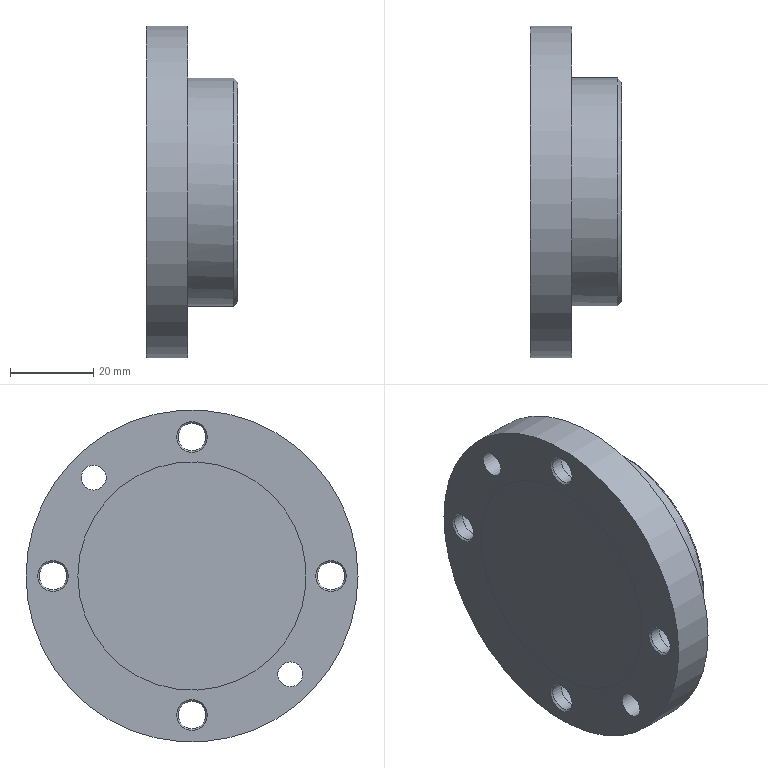Component | NX | LOCATING_BLOCK | 2 solids | 30 faces | volume 75084 mm3 | cylinder 13 | cone 9 | plane 8 | commonest cylinder face diameters 6.6 x4 11 x4 55 x2 6 x2 80 x1